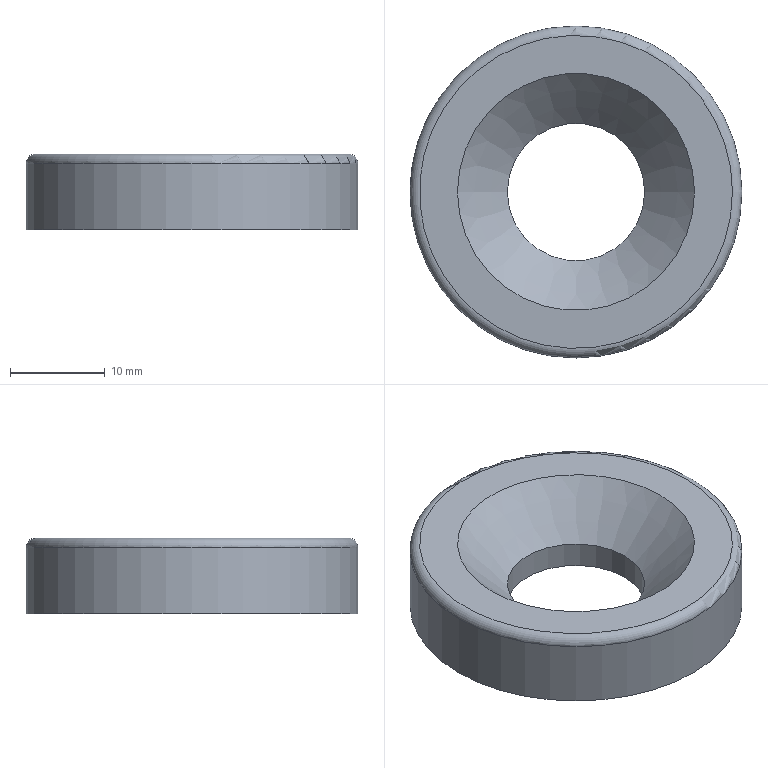Component | NX | SP_WASHER | 1 solid | 6 faces | box 35 x 35 x 8 mm | volume 5573 mm3 | cylinder 2 | plane 2 | cone 1 | torus 1 | commonest cylinder face diameters 14.5 x1 35 x1
STEP:
#1=CARTESIAN_POINT('',(0.,0.,0.));
#2=DIRECTION('',(0.,0.,1.));
#3=DIRECTION('',(1.,0.,0.));
#4=AXIS2_PLACEMENT_3D('',#1,#2,#3);
#5=CARTESIAN_POINT('',(-7.25,240.,315.75));
#6=VERTEX_POINT('',#5);
#7=CARTESIAN_POINT('',(0.,240.,315.75));
#8=DIRECTION('',(0.,0.,-1.));
#9=DIRECTION('',(-1.,0.,0.));
#10=AXIS2_PLACEMENT_3D('',#7,#8,#9);
#11=CIRCLE('',#10,7.25);
#12=CARTESIAN_POINT('',(0.,240.,321.));
#13=DIRECTION('',(0.,0.,1.));
#14=DIRECTION('',(1.,0.,0.));
#15=AXIS2_PLACEMENT_3D('',#12,#13,#14);
#16=CONICAL_SURFACE('',#15,12.5,0.7854);
#17=CARTESIAN_POINT('',(9.425,-5.25));
#18=DIRECTION('',(-1.,0.));
#19=VECTOR('',#18,1.);
#20=LINE('',#17,#19);
#21=(GEOMETRIC_REPRESENTATION_CONTEXT(2)PARAMETRIC_REPRESENTATION_CONTEXT()REPRESENTATION_CONTEXT('',''));
#22=DEFINITIONAL_REPRESENTATION('',(#20),#21);
#23=PCURVE('',#16,#22);
#24=CARTESIAN_POINT('',(0.,240.,313.));
#25=DIRECTION('',(0.,0.,-1.));
#26=DIRECTION('',(-1.,0.,0.));
#27=AXIS2_PLACEMENT_3D('',#24,#25,#26);
#28=CYLINDRICAL_SURFACE('',#27,7.25);
#29=CARTESIAN_POINT('',(0.,-2.75));
#30=DIRECTION('',(1.,0.));
#31=VECTOR('',#30,1.);
#32=LINE('',#29,#31);
#33=(GEOMETRIC_REPRESENTATION_CONTEXT(2)PARAMETRIC_REPRESENTATION_CONTEXT()REPRESENTATION_CONTEXT('',''));
#34=DEFINITIONAL_REPRESENTATION('',(#32),#33);
#35=PCURVE('',#28,#34);
#36=SURFACE_CURVE('',#11,(#23,#35),.PCURVE_S1.);
#37=EDGE_CURVE('',#6,#6,#36,.T.);
#38=ORIENTED_EDGE('',*,*,#37,.F.);
#39=CARTESIAN_POINT('',(-12.5,240.,321.));
#40=VERTEX_POINT('',#39);
#41=CARTESIAN_POINT('',(-7.25,240.,315.75));
#42=CARTESIAN_POINT('',(-12.5,240.,321.));
#43=B_SPLINE_CURVE_WITH_KNOTS('',1,(#41,#42),.UNSPECIFIED.,.F.,.F.,(2,2),(-7.425,0.),.PIECEWISE_BEZIER_KNOTS.);
#44=CARTESIAN_POINT('',(9.425,0.));
#45=DIRECTION('',(0.,1.));
#46=VECTOR('',#45,1.);
#47=LINE('',#44,#46);
#48=(GEOMETRIC_REPRESENTATION_CONTEXT(2)PARAMETRIC_REPRESENTATION_CONTEXT()REPRESENTATION_CONTEXT('',''));
#49=DEFINITIONAL_REPRESENTATION('',(#47),#48);
#50=PCURVE('',#16,#49);
#51=CARTESIAN_POINT('',(3.142,0.));
#52=DIRECTION('',(0.,1.));
#53=VECTOR('',#52,1.);
#54=LINE('',#51,#53);
#55=(GEOMETRIC_REPRESENTATION_CONTEXT(2)PARAMETRIC_REPRESENTATION_CONTEXT()REPRESENTATION_CONTEXT('',''));
#56=DEFINITIONAL_REPRESENTATION('',(#54),#55);
#57=PCURVE('',#16,#56);
#58=SEAM_CURVE('',#43,(#50,#57),.PCURVE_S1.);
#59=EDGE_CURVE('',#6,#40,#58,.T.);
#60=ORIENTED_EDGE('',*,*,#59,.T.);
#61=CARTESIAN_POINT('',(0.,240.,321.));
#62=DIRECTION('',(0.,0.,-1.));
#63=DIRECTION('',(-1.,0.,0.));
#64=AXIS2_PLACEMENT_3D('',#61,#62,#63);
#65=CIRCLE('',#64,12.5);
#66=CARTESIAN_POINT('',(9.425,0.));
#67=DIRECTION('',(-1.,0.));
#68=VECTOR('',#67,1.);
#69=LINE('',#66,#68);
#70=(GEOMETRIC_REPRESENTATION_CONTEXT(2)PARAMETRIC_REPRESENTATION_CONTEXT()REPRESENTATION_CONTEXT('',''));
#71=DEFINITIONAL_REPRESENTATION('',(#69),#70);
#72=PCURVE('',#16,#71);
#73=CARTESIAN_POINT('',(0.,257.5,321.));
#74=DIRECTION('',(0.,0.,1.));
#75=DIRECTION('',(1.,0.,0.));
#76=AXIS2_PLACEMENT_3D('',#73,#74,#75);
#77=PLANE('',#76);
#78=CARTESIAN_POINT('',(-12.5,-17.5));
#79=CARTESIAN_POINT('',(-12.5,4.151));
#80=CARTESIAN_POINT('',(6.25,-6.675));
#81=CARTESIAN_POINT('',(25.,-17.5));
#82=CARTESIAN_POINT('',(6.25,-28.325));
#83=CARTESIAN_POINT('',(-12.5,-39.151));
#84=CARTESIAN_POINT('',(-12.5,-17.5));
#85=(BOUNDED_CURVE()B_SPLINE_CURVE(2,(#78,#79,#80,#81,#82,#83,#84),.UNSPECIFIED.,.T.,.F.)B_SPLINE_CURVE_WITH_KNOTS((1,2,2,2,2,1),(-2.094,0.,2.094,4.189,6.283,8.378),.UNSPECIFIED.)CURVE()GEOMETRIC_REPRESENTATION_ITEM()RATIONAL_B_SPLINE_CURVE((1.,0.5,1.,0.5,1.,0.5,1.))REPRESENTATION_ITEM(''));
#86=(GEOMETRIC_REPRESENTATION_CONTEXT(2)PARAMETRIC_REPRESENTATION_CONTEXT()REPRESENTATION_CONTEXT('',''));
#87=DEFINITIONAL_REPRESENTATION('',(#85),#86);
#88=PCURVE('',#77,#87);
#89=SURFACE_CURVE('',#65,(#72,#88),.PCURVE_S1.);
#90=EDGE_CURVE('',#40,#40,#89,.T.);
#91=ORIENTED_EDGE('',*,*,#90,.T.);
#92=ORIENTED_EDGE('',*,*,#59,.F.);
#93=EDGE_LOOP('',(#38,#60,#91,#92));
#94=FACE_BOUND('',#93,.F.);
#95=ADVANCED_FACE('',(#94),#16,.F.);
#96=CARTESIAN_POINT('',(-7.25,240.,313.));
#97=VERTEX_POINT('',#96);
#98=CARTESIAN_POINT('',(0.,240.,313.));
#99=DIRECTION('',(0.,0.,-1.));
#100=DIRECTION('',(-1.,0.,0.));
#101=AXIS2_PLACEMENT_3D('',#98,#99,#100);
#102=CIRCLE('',#101,7.25);
#103=CARTESIAN_POINT('',(0.,0.));
#104=DIRECTION('',(1.,0.));
#105=VECTOR('',#104,1.);
#106=LINE('',#103,#105);
#107=(GEOMETRIC_REPRESENTATION_CONTEXT(2)PARAMETRIC_REPRESENTATION_CONTEXT()REPRESENTATION_CONTEXT('',''));
#108=DEFINITIONAL_REPRESENTATION('',(#106),#107);
#109=PCURVE('',#28,#108);
#110=CARTESIAN_POINT('',(0.,247.25,313.));
#111=DIRECTION('',(0.,0.,-1.));
#112=DIRECTION('',(-1.,0.,0.));
#113=AXIS2_PLACEMENT_3D('',#110,#111,#112);
#114=PLANE('',#113);
#115=CARTESIAN_POINT('',(0.,-7.25));
#116=DIRECTION('',(1.,0.));
#117=AXIS2_PLACEMENT_2D('',#115,#116);
#118=CIRCLE('',#117,7.25);
#119=(GEOMETRIC_REPRESENTATION_CONTEXT(2)PARAMETRIC_REPRESENTATION_CONTEXT()REPRESENTATION_CONTEXT('',''));
#120=DEFINITIONAL_REPRESENTATION('',(#118),#119);
#121=PCURVE('',#114,#120);
#122=SURFACE_CURVE('',#102,(#109,#121),.PCURVE_S1.);
#123=EDGE_CURVE('',#97,#97,#122,.T.);
#124=ORIENTED_EDGE('',*,*,#123,.F.);
#125=CARTESIAN_POINT('',(-7.25,240.,315.75));
#126=CARTESIAN_POINT('',(-7.25,240.,313.));
#127=B_SPLINE_CURVE_WITH_KNOTS('',1,(#125,#126),.UNSPECIFIED.,.F.,.F.,(2,2),(-2.75,0.),.PIECEWISE_BEZIER_KNOTS.);
#128=CARTESIAN_POINT('',(0.,0.));
#129=DIRECTION('',(0.,1.));
#130=VECTOR('',#129,1.);
#131=LINE('',#128,#130);
#132=(GEOMETRIC_REPRESENTATION_CONTEXT(2)PARAMETRIC_REPRESENTATION_CONTEXT()REPRESENTATION_CONTEXT('',''));
#133=DEFINITIONAL_REPRESENTATION('',(#131),#132);
#134=PCURVE('',#28,#133);
#135=CARTESIAN_POINT('',(6.283,0.));
#136=DIRECTION('',(0.,1.));
#137=VECTOR('',#136,1.);
#138=LINE('',#135,#137);
#139=(GEOMETRIC_REPRESENTATION_CONTEXT(2)PARAMETRIC_REPRESENTATION_CONTEXT()REPRESENTATION_CONTEXT('',''));
#140=DEFINITIONAL_REPRESENTATION('',(#138),#139);
#141=PCURVE('',#28,#140);
#142=SEAM_CURVE('',#127,(#134,#141),.PCURVE_S1.);
#143=EDGE_CURVE('',#6,#97,#142,.T.);
#144=ORIENTED_EDGE('',*,*,#143,.F.);
#145=ORIENTED_EDGE('',*,*,#37,.T.);
#146=ORIENTED_EDGE('',*,*,#143,.T.);
#147=EDGE_LOOP('',(#124,#144,#145,#146));
#148=FACE_BOUND('',#147,.F.);
#149=ADVANCED_FACE('',(#148),#28,.F.);
#150=CARTESIAN_POINT('',(-17.5,240.,313.));
#151=VERTEX_POINT('',#150);
#152=CARTESIAN_POINT('',(0.,240.,313.));
#153=DIRECTION('',(0.,0.,-1.));
#154=DIRECTION('',(-1.,0.,0.));
#155=AXIS2_PLACEMENT_3D('',#152,#153,#154);
#156=CIRCLE('',#155,17.5);
#157=CARTESIAN_POINT('',(0.,-7.25));
#158=DIRECTION('',(1.,0.));
#159=AXIS2_PLACEMENT_2D('',#157,#158);
#160=CIRCLE('',#159,17.5);
#161=(GEOMETRIC_REPRESENTATION_CONTEXT(2)PARAMETRIC_REPRESENTATION_CONTEXT()REPRESENTATION_CONTEXT('',''));
#162=DEFINITIONAL_REPRESENTATION('',(#160),#161);
#163=PCURVE('',#114,#162);
#164=CARTESIAN_POINT('',(0.,240.,313.));
#165=DIRECTION('',(0.,0.,-1.));
#166=DIRECTION('',(-1.,0.,0.));
#167=AXIS2_PLACEMENT_3D('',#164,#165,#166);
#168=CYLINDRICAL_SURFACE('',#167,17.5);
#169=CARTESIAN_POINT('',(0.,0.));
#170=DIRECTION('',(1.,0.));
#171=VECTOR('',#170,1.);
#172=LINE('',#169,#171);
#173=(GEOMETRIC_REPRESENTATION_CONTEXT(2)PARAMETRIC_REPRESENTATION_CONTEXT()REPRESENTATION_CONTEXT('',''));
#174=DEFINITIONAL_REPRESENTATION('',(#172),#173);
#175=PCURVE('',#168,#174);
#176=SURFACE_CURVE('',#156,(#163,#175),.PCURVE_S1.);
#177=EDGE_CURVE('',#151,#151,#176,.T.);
#178=ORIENTED_EDGE('',*,*,#177,.T.);
#179=EDGE_LOOP('',(#178));
#180=FACE_BOUND('',#179,.T.);
#181=ORIENTED_EDGE('',*,*,#123,.F.);
#182=EDGE_LOOP('',(#181));
#183=FACE_BOUND('',#182,.T.);
#184=ADVANCED_FACE('',(#180,#183),#114,.T.);
#185=CARTESIAN_POINT('',(17.5,240.,320.));
#186=VERTEX_POINT('',#185);
#187=CARTESIAN_POINT('',(-17.5,240.,320.));
#188=VERTEX_POINT('',#187);
#189=CARTESIAN_POINT('',(0.,240.,320.));
#190=DIRECTION('',(0.,0.,-1.));
#191=DIRECTION('',(1.,0.,0.));
#192=AXIS2_PLACEMENT_3D('',#189,#190,#191);
#193=CIRCLE('',#192,17.5);
#194=CARTESIAN_POINT('',(3.142,-7.));
#195=DIRECTION('',(1.,0.));
#196=VECTOR('',#195,1.);
#197=LINE('',#194,#196);
#198=(GEOMETRIC_REPRESENTATION_CONTEXT(2)PARAMETRIC_REPRESENTATION_CONTEXT()REPRESENTATION_CONTEXT('',''));
#199=DEFINITIONAL_REPRESENTATION('',(#197),#198);
#200=PCURVE('',#168,#199);
#201=CARTESIAN_POINT('',(0.,240.,320.));
#202=DIRECTION('',(0.,0.,1.));
#203=DIRECTION('',(1.,0.,0.));
#204=AXIS2_PLACEMENT_3D('',#201,#202,#203);
#205=TOROIDAL_SURFACE('',#204,16.5,1.);
#206=CARTESIAN_POINT('',(6.283,6.283));
#207=DIRECTION('',(-1.,0.));
#208=VECTOR('',#207,1.);
#209=LINE('',#206,#208);
#210=(GEOMETRIC_REPRESENTATION_CONTEXT(2)PARAMETRIC_REPRESENTATION_CONTEXT()REPRESENTATION_CONTEXT('',''));
#211=DEFINITIONAL_REPRESENTATION('',(#209),#210);
#212=PCURVE('',#205,#211);
#213=SURFACE_CURVE('',#193,(#200,#212),.PCURVE_S1.);
#214=EDGE_CURVE('',#186,#188,#213,.T.);
#215=ORIENTED_EDGE('',*,*,#214,.T.);
#216=CARTESIAN_POINT('',(-17.5,240.,320.));
#217=CARTESIAN_POINT('',(-17.5,240.,313.));
#218=B_SPLINE_CURVE_WITH_KNOTS('',1,(#216,#217),.UNSPECIFIED.,.F.,.F.,(2,2),(-7.,0.),.PIECEWISE_BEZIER_KNOTS.);
#219=CARTESIAN_POINT('',(6.283,0.));
#220=DIRECTION('',(0.,1.));
#221=VECTOR('',#220,1.);
#222=LINE('',#219,#221);
#223=(GEOMETRIC_REPRESENTATION_CONTEXT(2)PARAMETRIC_REPRESENTATION_CONTEXT()REPRESENTATION_CONTEXT('',''));
#224=DEFINITIONAL_REPRESENTATION('',(#222),#223);
#225=PCURVE('',#168,#224);
#226=CARTESIAN_POINT('',(0.,0.));
#227=DIRECTION('',(0.,1.));
#228=VECTOR('',#227,1.);
#229=LINE('',#226,#228);
#230=(GEOMETRIC_REPRESENTATION_CONTEXT(2)PARAMETRIC_REPRESENTATION_CONTEXT()REPRESENTATION_CONTEXT('',''));
#231=DEFINITIONAL_REPRESENTATION('',(#229),#230);
#232=PCURVE('',#168,#231);
#233=SEAM_CURVE('',#218,(#225,#232),.PCURVE_S1.);
#234=EDGE_CURVE('',#188,#151,#233,.T.);
#235=ORIENTED_EDGE('',*,*,#234,.T.);
#236=ORIENTED_EDGE('',*,*,#177,.F.);
#237=ORIENTED_EDGE('',*,*,#234,.F.);
#238=CARTESIAN_POINT('',(0.,240.,320.));
#239=DIRECTION('',(0.,0.,-1.));
#240=DIRECTION('',(1.,0.,0.));
#241=AXIS2_PLACEMENT_3D('',#238,#239,#240);
#242=CIRCLE('',#241,17.5);
#243=CARTESIAN_POINT('',(-3.142,-7.));
#244=DIRECTION('',(1.,0.));
#245=VECTOR('',#244,1.);
#246=LINE('',#243,#245);
#247=(GEOMETRIC_REPRESENTATION_CONTEXT(2)PARAMETRIC_REPRESENTATION_CONTEXT()REPRESENTATION_CONTEXT('',''));
#248=DEFINITIONAL_REPRESENTATION('',(#246),#247);
#249=PCURVE('',#168,#248);
#250=CARTESIAN_POINT('',(6.283,6.283));
#251=DIRECTION('',(-1.,0.));
#252=VECTOR('',#251,1.);
#253=LINE('',#250,#252);
#254=(GEOMETRIC_REPRESENTATION_CONTEXT(2)PARAMETRIC_REPRESENTATION_CONTEXT()REPRESENTATION_CONTEXT('',''));
#255=DEFINITIONAL_REPRESENTATION('',(#253),#254);
#256=PCURVE('',#205,#255);
#257=SURFACE_CURVE('',#242,(#249,#256),.PCURVE_S1.);
#258=EDGE_CURVE('',#188,#186,#257,.T.);
#259=ORIENTED_EDGE('',*,*,#258,.T.);
#260=EDGE_LOOP('',(#215,#235,#236,#237,#259));
#261=FACE_BOUND('',#260,.T.);
#262=ADVANCED_FACE('',(#261),#168,.T.);
#263=CARTESIAN_POINT('',(16.5,240.,321.));
#264=VERTEX_POINT('',#263);
#265=CARTESIAN_POINT('',(0.,240.,321.));
#266=DIRECTION('',(0.,0.,1.));
#267=DIRECTION('',(1.,0.,0.));
#268=AXIS2_PLACEMENT_3D('',#265,#266,#267);
#269=CIRCLE('',#268,16.5);
#270=CARTESIAN_POINT('',(0.,-17.5));
#271=DIRECTION('',(1.,0.));
#272=AXIS2_PLACEMENT_2D('',#270,#271);
#273=CIRCLE('',#272,16.5);
#274=(GEOMETRIC_REPRESENTATION_CONTEXT(2)PARAMETRIC_REPRESENTATION_CONTEXT()REPRESENTATION_CONTEXT('',''));
#275=DEFINITIONAL_REPRESENTATION('',(#273),#274);
#276=PCURVE('',#77,#275);
#277=CARTESIAN_POINT('',(0.,7.854));
#278=DIRECTION('',(1.,0.));
#279=VECTOR('',#278,1.);
#280=LINE('',#277,#279);
#281=(GEOMETRIC_REPRESENTATION_CONTEXT(2)PARAMETRIC_REPRESENTATION_CONTEXT()REPRESENTATION_CONTEXT('',''));
#282=DEFINITIONAL_REPRESENTATION('',(#280),#281);
#283=PCURVE('',#205,#282);
#284=SURFACE_CURVE('',#269,(#276,#283),.PCURVE_S1.);
#285=EDGE_CURVE('',#264,#264,#284,.T.);
#286=ORIENTED_EDGE('',*,*,#285,.T.);
#287=EDGE_LOOP('',(#286));
#288=FACE_BOUND('',#287,.T.);
#289=ORIENTED_EDGE('',*,*,#90,.T.);
#290=EDGE_LOOP('',(#289));
#291=FACE_BOUND('',#290,.T.);
#292=ADVANCED_FACE('',(#288,#291),#77,.T.);
#293=ORIENTED_EDGE('',*,*,#285,.F.);
#294=CARTESIAN_POINT('',(17.5,240.,320.));
#295=CARTESIAN_POINT('',(17.5,240.,320.267));
#296=CARTESIAN_POINT('',(17.415,240.,320.528));
#297=CARTESIAN_POINT('',(17.252,240.,320.752));
#298=CARTESIAN_POINT('',(17.028,240.,320.915));
#299=CARTESIAN_POINT('',(16.767,240.,321.));
#300=CARTESIAN_POINT('',(16.5,240.,321.));
#301=(BOUNDED_CURVE()B_SPLINE_CURVE(6,(#294,#295,#296,#297,#298,#299,#300),.UNSPECIFIED.,.F.,.F.)B_SPLINE_CURVE_WITH_KNOTS((7,7),(0.,1.571),.PIECEWISE_BEZIER_KNOTS.)CURVE()GEOMETRIC_REPRESENTATION_ITEM()RATIONAL_B_SPLINE_CURVE((1.031,1.01,0.9979,0.994,0.9979,1.01,1.031))REPRESENTATION_ITEM(''));
#302=CARTESIAN_POINT('',(0.,6.283));
#303=DIRECTION('',(0.,1.));
#304=VECTOR('',#303,1.);
#305=LINE('',#302,#304);
#306=(GEOMETRIC_REPRESENTATION_CONTEXT(2)PARAMETRIC_REPRESENTATION_CONTEXT()REPRESENTATION_CONTEXT('',''));
#307=DEFINITIONAL_REPRESENTATION('',(#305),#306);
#308=PCURVE('',#205,#307);
#309=CARTESIAN_POINT('',(6.283,6.283));
#310=DIRECTION('',(0.,1.));
#311=VECTOR('',#310,1.);
#312=LINE('',#309,#311);
#313=(GEOMETRIC_REPRESENTATION_CONTEXT(2)PARAMETRIC_REPRESENTATION_CONTEXT()REPRESENTATION_CONTEXT('',''));
#314=DEFINITIONAL_REPRESENTATION('',(#312),#313);
#315=PCURVE('',#205,#314);
#316=SEAM_CURVE('',#301,(#308,#315),.PCURVE_S1.);
#317=EDGE_CURVE('',#186,#264,#316,.T.);
#318=ORIENTED_EDGE('',*,*,#317,.F.);
#319=ORIENTED_EDGE('',*,*,#258,.F.);
#320=ORIENTED_EDGE('',*,*,#214,.F.);
#321=ORIENTED_EDGE('',*,*,#317,.T.);
#322=EDGE_LOOP('',(#293,#318,#319,#320,#321));
#323=FACE_BOUND('',#322,.T.);
#324=ADVANCED_FACE('',(#323),#205,.T.);
#325=CLOSED_SHELL('',(#95,#149,#184,#262,#292,#324));
#326=MANIFOLD_SOLID_BREP('',#325);
#327=(LENGTH_UNIT()NAMED_UNIT(*)SI_UNIT(.MILLI.,.METRE.));
#328=UNCERTAINTY_MEASURE_WITH_UNIT(LENGTH_MEASURE(0.00001),#327,'','');
#329=(NAMED_UNIT(*)PLANE_ANGLE_UNIT()SI_UNIT($,.RADIAN.));
#330=(NAMED_UNIT(*)SI_UNIT($,.STERADIAN.)SOLID_ANGLE_UNIT());
#331=(GEOMETRIC_REPRESENTATION_CONTEXT(3)GLOBAL_UNCERTAINTY_ASSIGNED_CONTEXT((#328))GLOBAL_UNIT_ASSIGNED_CONTEXT((#327,#329,#330))REPRESENTATION_CONTEXT('',''));
#332=ADVANCED_BREP_SHAPE_REPRESENTATION('',(#4,#326),#331);